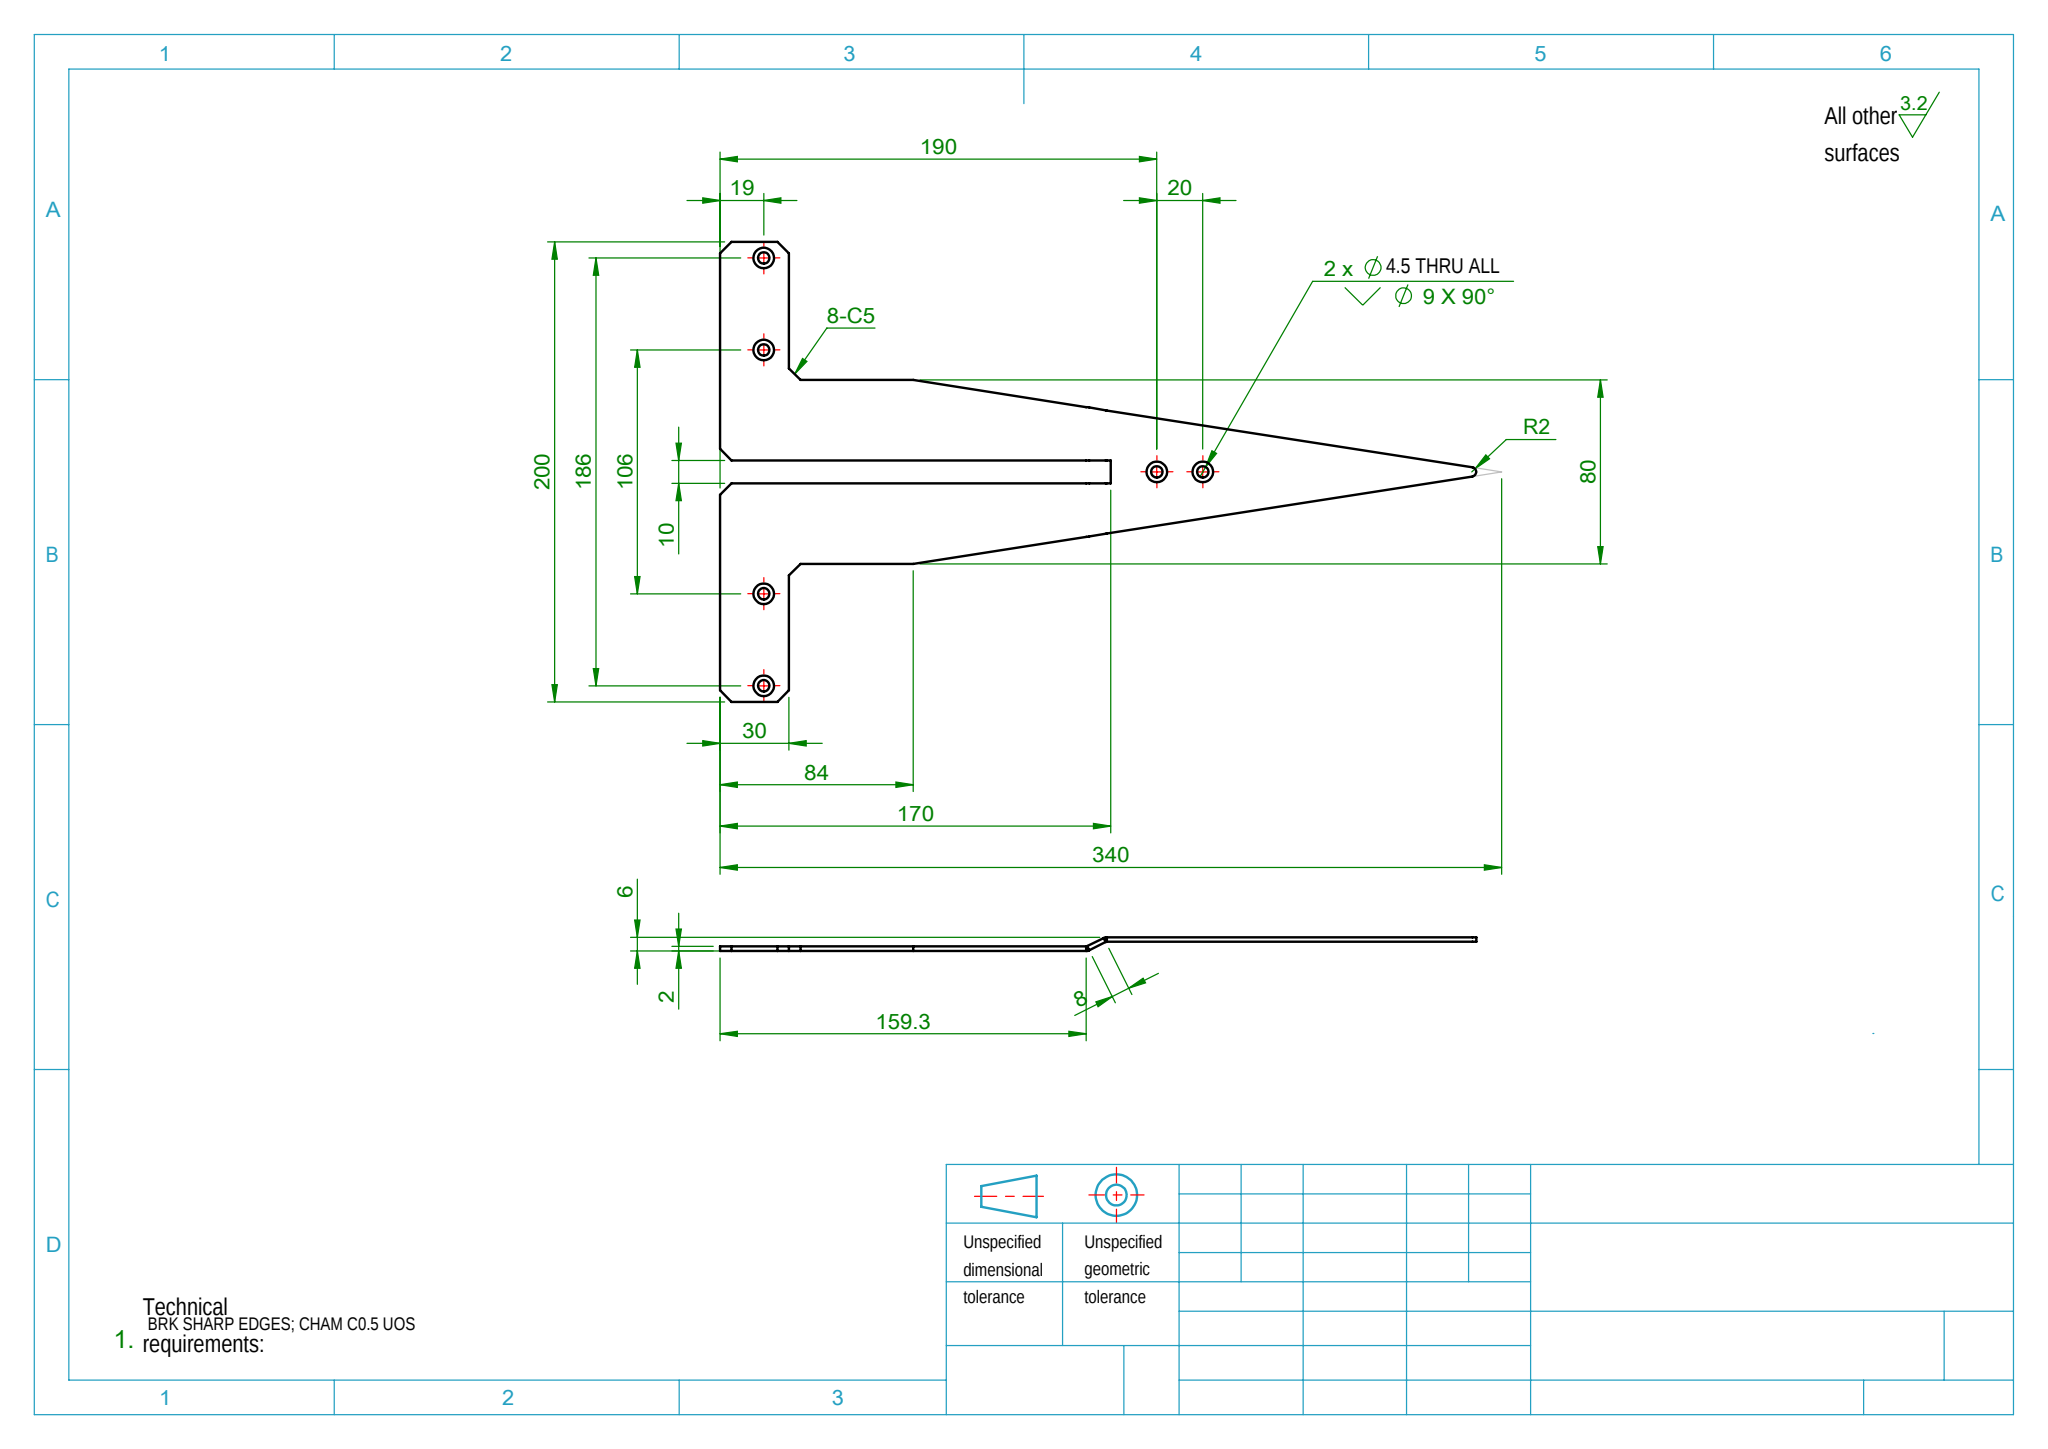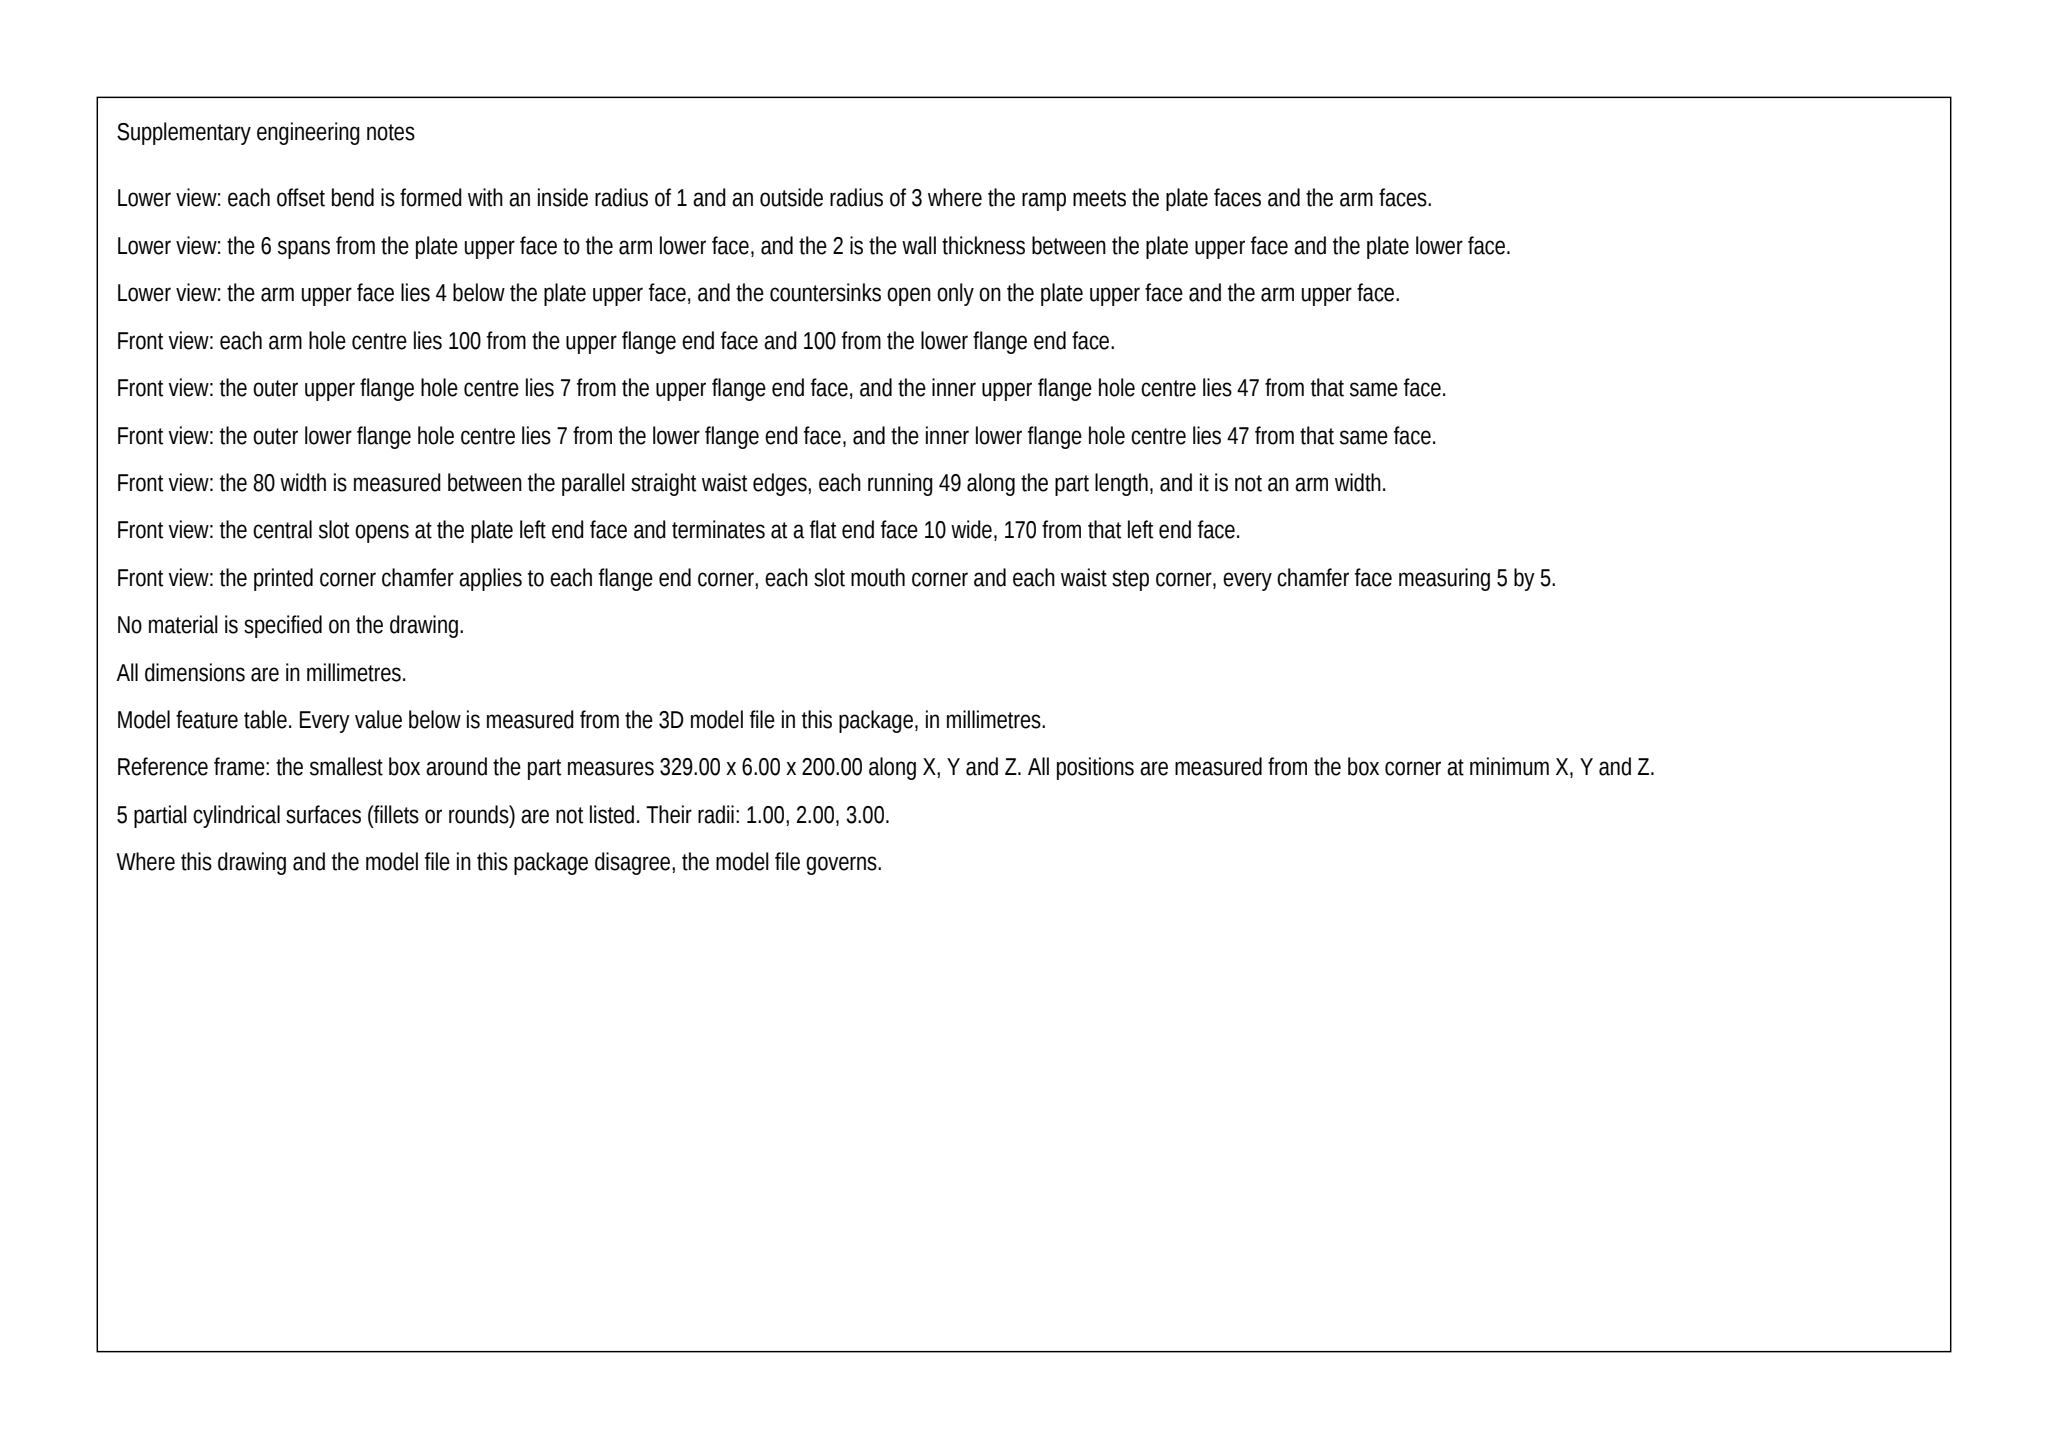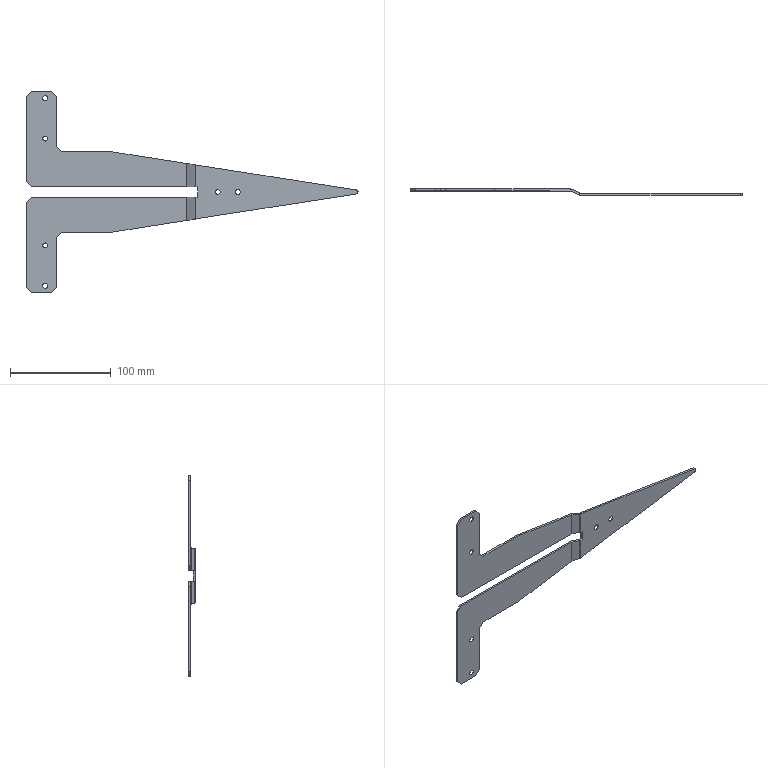Part | SolidWorks | mm | 1 solid | 68 faces | box 329 x 6 x 200 mm | volume 37150 mm3 | plane 43 | cone 12 | cylinder 9 | spline 4 | commonest cylinder face diameters 2 x4 6 x4 4 x1
Drawing notes:
4 X Ø4.5 THRU ALL IN FLANGE, CSK Ø9 X 90° BOTH SIDES | from the solid: cones[included_angle,ref_dia]=[90.0, 8.96] x12 = 6 holes csk both faces, same size as the 2 x Ø4.5 holes; plate thk 2 (y planes 0.02/2.02, 4.02/6.02)
JOGGLE BEND AT 159.3: R1 INSIDE, R3 OUTSIDE | from the solid: z-axis cyls Ø2.0 at x=159.29 & x=168.24 (inner, R1) and Ø6.0 at same x (outer, R3), y=3.02
2 X Ø4.5 CSK HOLES ON HORIZ CL, 100 FROM TOP & BTM EDGE | from the solid: bbox z=200; part symmetric about z=100 (z planes 95/105, 60/140, 0/200) and R2 tip cyl Ø4.0 axis y at z=100.01
2 X Ø4.5 THRU: CSK Ø9 X 90° BOTH SIDES | from the solid: cones[90.0, ref_dia 8.96] count 12 = 6 holes csk on both faces; Ø4.5 arm holes at x=159.29 & 168.24 each have csk on y=0.02 and y=6.02 faces